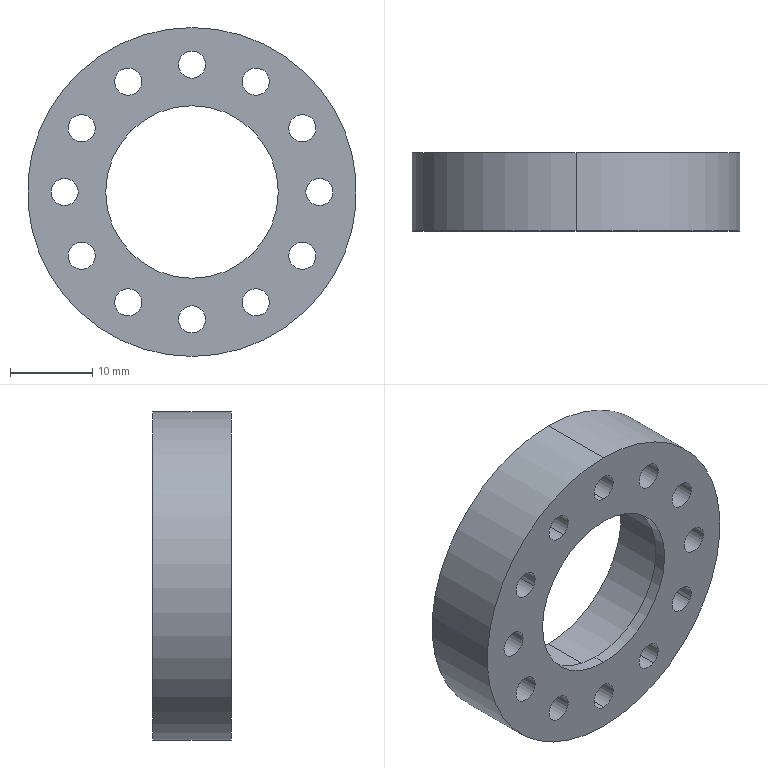Part | SolidWorks | mm | 1 solid | 33 faces | box 40 x 9.5 x 40 mm | volume 6516 mm3 | cylinder 30 | plane 3 | commonest cylinder face diameters 3.3 x24 21 x2 25 x2 40 x2
build123d program:
from build123d import *

# Parameters (mm, degrees)
SKETCH1_R           = 20
BOSS_EXTRUDE1_DEPTH = 9.5
SKETCH2_R           = 10
BOSS_EXTRUDE2_DEPTH = 7
SKETCH3_R           = 12.5
CUT_EXTRUDE1_DEPTH  = 8
SKETCH4_R           = 10.5
CUT_EXTRUDE2_DEPTH  = 30.394
M4_TAPPED_HOLE1_D   = 3.3
CIRPATTERN1_COUNT   = 12


with BuildPart() as part:
    # Sketch1 → Boss-Extrude1 (new body)
    with BuildSketch(Plane(origin=(0, 0, 0), x_dir=(1, 0, 0), z_dir=(0, 1, 0))):
        with Locations(Location((0, 0, 0), (0, 0, 270))):
            Circle(SKETCH1_R)
    extrude(amount=BOSS_EXTRUDE1_DEPTH)

    # Sketch2 → Boss-Extrude2 (add)
    with BuildSketch(Plane(origin=(0, 9.5, 0), x_dir=(1, 0, 0), z_dir=(0, 1, 0))):
        Circle(SKETCH2_R)
    extrude(amount=-BOSS_EXTRUDE2_DEPTH)

    # Sketch3 → Cut-Extrude1 (cut)
    with BuildSketch(Plane(origin=(0, 9.5, 0), x_dir=(1, 0, 0), z_dir=(0, 1, 0))):
        with Locations(Location((0, 0, 0), (0, 0, 270))):
            Circle(SKETCH3_R)
    extrude(amount=-CUT_EXTRUDE1_DEPTH, mode=Mode.SUBTRACT)

    # Sketch4 → Cut-Extrude2 (cut, through all)
    with BuildSketch(Plane(origin=(0, 1.5, 0), x_dir=(1, 0, 0), z_dir=(0, 1, 0))):
        with Locations(Location((0, 0, 0), (0, 0, 270))):
            Circle(SKETCH4_R)
    extrude(amount=-CUT_EXTRUDE2_DEPTH, mode=Mode.SUBTRACT)

    # M4 Tapped Hole1 (through all)
    with Locations(Plane(origin=(0, 0, 0), x_dir=(-1, 0, 0), z_dir=(0, -1, 0))):
        with Locations((0, -15.5)):
            m4_tapped_hole1 = Hole(M4_TAPPED_HOLE1_D / 2)

    # CirPattern1: M4 Tapped Hole1 ×12 about axis
    cirpattern1_axis = Axis((0, 0, 0), (0, 1, 0))
    for i in range(1, CIRPATTERN1_COUNT):
        add(m4_tapped_hole1.rotate(cirpattern1_axis, i * 360 / CIRPATTERN1_COUNT), mode=Mode.SUBTRACT)


solid = part.part
STEP:
#1=CARTESIAN_POINT('',(8.575,9.5,14.852));
#2=VERTEX_POINT('',#1);
#3=CARTESIAN_POINT('',(6.925,9.5,11.994));
#4=VERTEX_POINT('',#3);
#5=CARTESIAN_POINT('',(7.75,9.5,13.423));
#6=DIRECTION('',(0.,-1.,0.));
#7=DIRECTION('',(-0.5,0.,-0.866));
#8=AXIS2_PLACEMENT_3D('',#5,#6,#7);
#9=CIRCLE('',#8,1.65);
#10=EDGE_CURVE('',#2,#4,#9,.T.);
#11=ORIENTED_EDGE('',*,*,#10,.F.);
#12=CARTESIAN_POINT('',(8.575,-0.,14.852));
#13=VERTEX_POINT('',#12);
#14=CARTESIAN_POINT('',(8.575,0.,14.852));
#15=DIRECTION('',(0.,-1.,0.));
#16=VECTOR('',#15,1000.);
#17=LINE('',#14,#16);
#18=EDGE_CURVE('',#2,#13,#17,.T.);
#19=ORIENTED_EDGE('',*,*,#18,.T.);
#20=CARTESIAN_POINT('',(6.925,-0.,11.994));
#21=VERTEX_POINT('',#20);
#22=CARTESIAN_POINT('',(7.75,-0.,13.423));
#23=DIRECTION('',(0.,-1.,0.));
#24=DIRECTION('',(-0.5,0.,-0.866));
#25=AXIS2_PLACEMENT_3D('',#22,#23,#24);
#26=CIRCLE('',#25,1.65);
#27=EDGE_CURVE('',#13,#21,#26,.T.);
#28=ORIENTED_EDGE('',*,*,#27,.T.);
#29=CARTESIAN_POINT('',(6.925,0.,11.994));
#30=DIRECTION('',(0.,-1.,0.));
#31=VECTOR('',#30,1000.);
#32=LINE('',#29,#31);
#33=EDGE_CURVE('',#4,#21,#32,.T.);
#34=ORIENTED_EDGE('',*,*,#33,.F.);
#35=EDGE_LOOP('',(#11,#19,#28,#34));
#36=FACE_OUTER_BOUND('',#35,.T.);
#37=CARTESIAN_POINT('',(7.75,0.,13.423));
#38=DIRECTION('',(0.,-1.,0.));
#39=DIRECTION('',(-0.5,0.,-0.866));
#40=AXIS2_PLACEMENT_3D('',#37,#38,#39);
#41=CYLINDRICAL_SURFACE('',#40,1.65);
#42=ADVANCED_FACE('',(#36),#41,.F.);
#43=CARTESIAN_POINT('',(14.852,9.5,8.575));
#44=VERTEX_POINT('',#43);
#45=CARTESIAN_POINT('',(11.994,9.5,6.925));
#46=VERTEX_POINT('',#45);
#47=CARTESIAN_POINT('',(13.423,9.5,7.75));
#48=DIRECTION('',(0.,-1.,0.));
#49=DIRECTION('',(-0.866,0.,-0.5));
#50=AXIS2_PLACEMENT_3D('',#47,#48,#49);
#51=CIRCLE('',#50,1.65);
#52=EDGE_CURVE('',#44,#46,#51,.T.);
#53=ORIENTED_EDGE('',*,*,#52,.F.);
#54=CARTESIAN_POINT('',(14.852,-0.,8.575));
#55=VERTEX_POINT('',#54);
#56=CARTESIAN_POINT('',(14.852,0.,8.575));
#57=DIRECTION('',(0.,-1.,0.));
#58=VECTOR('',#57,1000.);
#59=LINE('',#56,#58);
#60=EDGE_CURVE('',#44,#55,#59,.T.);
#61=ORIENTED_EDGE('',*,*,#60,.T.);
#62=CARTESIAN_POINT('',(11.994,-0.,6.925));
#63=VERTEX_POINT('',#62);
#64=CARTESIAN_POINT('',(13.423,-0.,7.75));
#65=DIRECTION('',(0.,-1.,0.));
#66=DIRECTION('',(-0.866,0.,-0.5));
#67=AXIS2_PLACEMENT_3D('',#64,#65,#66);
#68=CIRCLE('',#67,1.65);
#69=EDGE_CURVE('',#55,#63,#68,.T.);
#70=ORIENTED_EDGE('',*,*,#69,.T.);
#71=CARTESIAN_POINT('',(11.994,0.,6.925));
#72=DIRECTION('',(0.,-1.,0.));
#73=VECTOR('',#72,1000.);
#74=LINE('',#71,#73);
#75=EDGE_CURVE('',#46,#63,#74,.T.);
#76=ORIENTED_EDGE('',*,*,#75,.F.);
#77=EDGE_LOOP('',(#53,#61,#70,#76));
#78=FACE_OUTER_BOUND('',#77,.T.);
#79=CARTESIAN_POINT('',(13.423,0.,7.75));
#80=DIRECTION('',(0.,-1.,0.));
#81=DIRECTION('',(-0.866,0.,-0.5));
#82=AXIS2_PLACEMENT_3D('',#79,#80,#81);
#83=CYLINDRICAL_SURFACE('',#82,1.65);
#84=ADVANCED_FACE('',(#78),#83,.F.);
#85=CARTESIAN_POINT('',(17.15,9.5,0.));
#86=VERTEX_POINT('',#85);
#87=CARTESIAN_POINT('',(13.85,9.5,0.));
#88=VERTEX_POINT('',#87);
#89=CARTESIAN_POINT('',(15.5,9.5,0.));
#90=DIRECTION('',(0.,-1.,0.));
#91=DIRECTION('',(-1.,0.,-0.));
#92=AXIS2_PLACEMENT_3D('',#89,#90,#91);
#93=CIRCLE('',#92,1.65);
#94=EDGE_CURVE('',#86,#88,#93,.T.);
#95=ORIENTED_EDGE('',*,*,#94,.F.);
#96=CARTESIAN_POINT('',(17.15,-0.,0.));
#97=VERTEX_POINT('',#96);
#98=CARTESIAN_POINT('',(17.15,0.,0.));
#99=DIRECTION('',(0.,-1.,0.));
#100=VECTOR('',#99,1000.);
#101=LINE('',#98,#100);
#102=EDGE_CURVE('',#86,#97,#101,.T.);
#103=ORIENTED_EDGE('',*,*,#102,.T.);
#104=CARTESIAN_POINT('',(13.85,-0.,0.));
#105=VERTEX_POINT('',#104);
#106=CARTESIAN_POINT('',(15.5,-0.,0.));
#107=DIRECTION('',(0.,-1.,0.));
#108=DIRECTION('',(-1.,0.,-0.));
#109=AXIS2_PLACEMENT_3D('',#106,#107,#108);
#110=CIRCLE('',#109,1.65);
#111=EDGE_CURVE('',#97,#105,#110,.T.);
#112=ORIENTED_EDGE('',*,*,#111,.T.);
#113=CARTESIAN_POINT('',(13.85,0.,0.));
#114=DIRECTION('',(0.,-1.,0.));
#115=VECTOR('',#114,1000.);
#116=LINE('',#113,#115);
#117=EDGE_CURVE('',#88,#105,#116,.T.);
#118=ORIENTED_EDGE('',*,*,#117,.F.);
#119=EDGE_LOOP('',(#95,#103,#112,#118));
#120=FACE_OUTER_BOUND('',#119,.T.);
#121=CARTESIAN_POINT('',(15.5,0.,0.));
#122=DIRECTION('',(0.,-1.,0.));
#123=DIRECTION('',(-1.,0.,-0.));
#124=AXIS2_PLACEMENT_3D('',#121,#122,#123);
#125=CYLINDRICAL_SURFACE('',#124,1.65);
#126=ADVANCED_FACE('',(#120),#125,.F.);
#127=CARTESIAN_POINT('',(14.852,9.5,-8.575));
#128=VERTEX_POINT('',#127);
#129=CARTESIAN_POINT('',(11.994,9.5,-6.925));
#130=VERTEX_POINT('',#129);
#131=CARTESIAN_POINT('',(13.423,9.5,-7.75));
#132=DIRECTION('',(0.,-1.,0.));
#133=DIRECTION('',(-0.866,0.,0.5));
#134=AXIS2_PLACEMENT_3D('',#131,#132,#133);
#135=CIRCLE('',#134,1.65);
#136=EDGE_CURVE('',#128,#130,#135,.T.);
#137=ORIENTED_EDGE('',*,*,#136,.F.);
#138=CARTESIAN_POINT('',(14.852,-0.,-8.575));
#139=VERTEX_POINT('',#138);
#140=CARTESIAN_POINT('',(14.852,0.,-8.575));
#141=DIRECTION('',(0.,-1.,0.));
#142=VECTOR('',#141,1000.);
#143=LINE('',#140,#142);
#144=EDGE_CURVE('',#128,#139,#143,.T.);
#145=ORIENTED_EDGE('',*,*,#144,.T.);
#146=CARTESIAN_POINT('',(11.994,-0.,-6.925));
#147=VERTEX_POINT('',#146);
#148=CARTESIAN_POINT('',(13.423,-0.,-7.75));
#149=DIRECTION('',(0.,-1.,0.));
#150=DIRECTION('',(-0.866,0.,0.5));
#151=AXIS2_PLACEMENT_3D('',#148,#149,#150);
#152=CIRCLE('',#151,1.65);
#153=EDGE_CURVE('',#139,#147,#152,.T.);
#154=ORIENTED_EDGE('',*,*,#153,.T.);
#155=CARTESIAN_POINT('',(11.994,0.,-6.925));
#156=DIRECTION('',(0.,-1.,0.));
#157=VECTOR('',#156,1000.);
#158=LINE('',#155,#157);
#159=EDGE_CURVE('',#130,#147,#158,.T.);
#160=ORIENTED_EDGE('',*,*,#159,.F.);
#161=EDGE_LOOP('',(#137,#145,#154,#160));
#162=FACE_OUTER_BOUND('',#161,.T.);
#163=CARTESIAN_POINT('',(13.423,0.,-7.75));
#164=DIRECTION('',(0.,-1.,0.));
#165=DIRECTION('',(-0.866,0.,0.5));
#166=AXIS2_PLACEMENT_3D('',#163,#164,#165);
#167=CYLINDRICAL_SURFACE('',#166,1.65);
#168=ADVANCED_FACE('',(#162),#167,.F.);
#169=CARTESIAN_POINT('',(8.575,9.5,-14.852));
#170=VERTEX_POINT('',#169);
#171=CARTESIAN_POINT('',(6.925,9.5,-11.994));
#172=VERTEX_POINT('',#171);
#173=CARTESIAN_POINT('',(7.75,9.5,-13.423));
#174=DIRECTION('',(0.,-1.,0.));
#175=DIRECTION('',(-0.5,0.,0.866));
#176=AXIS2_PLACEMENT_3D('',#173,#174,#175);
#177=CIRCLE('',#176,1.65);
#178=EDGE_CURVE('',#170,#172,#177,.T.);
#179=ORIENTED_EDGE('',*,*,#178,.F.);
#180=CARTESIAN_POINT('',(8.575,-0.,-14.852));
#181=VERTEX_POINT('',#180);
#182=CARTESIAN_POINT('',(8.575,0.,-14.852));
#183=DIRECTION('',(0.,-1.,0.));
#184=VECTOR('',#183,1000.);
#185=LINE('',#182,#184);
#186=EDGE_CURVE('',#170,#181,#185,.T.);
#187=ORIENTED_EDGE('',*,*,#186,.T.);
#188=CARTESIAN_POINT('',(6.925,-0.,-11.994));
#189=VERTEX_POINT('',#188);
#190=CARTESIAN_POINT('',(7.75,-0.,-13.423));
#191=DIRECTION('',(0.,-1.,0.));
#192=DIRECTION('',(-0.5,0.,0.866));
#193=AXIS2_PLACEMENT_3D('',#190,#191,#192);
#194=CIRCLE('',#193,1.65);
#195=EDGE_CURVE('',#181,#189,#194,.T.);
#196=ORIENTED_EDGE('',*,*,#195,.T.);
#197=CARTESIAN_POINT('',(6.925,0.,-11.994));
#198=DIRECTION('',(0.,-1.,0.));
#199=VECTOR('',#198,1000.);
#200=LINE('',#197,#199);
#201=EDGE_CURVE('',#172,#189,#200,.T.);
#202=ORIENTED_EDGE('',*,*,#201,.F.);
#203=EDGE_LOOP('',(#179,#187,#196,#202));
#204=FACE_OUTER_BOUND('',#203,.T.);
#205=CARTESIAN_POINT('',(7.75,0.,-13.423));
#206=DIRECTION('',(0.,-1.,0.));
#207=DIRECTION('',(-0.5,0.,0.866));
#208=AXIS2_PLACEMENT_3D('',#205,#206,#207);
#209=CYLINDRICAL_SURFACE('',#208,1.65);
#210=ADVANCED_FACE('',(#204),#209,.F.);
#211=CARTESIAN_POINT('',(0.,9.5,-17.15));
#212=VERTEX_POINT('',#211);
#213=CARTESIAN_POINT('',(0.,9.5,-13.85));
#214=VERTEX_POINT('',#213);
#215=CARTESIAN_POINT('',(0.,9.5,-15.5));
#216=DIRECTION('',(0.,-1.,0.));
#217=DIRECTION('',(0.,0.,1.));
#218=AXIS2_PLACEMENT_3D('',#215,#216,#217);
#219=CIRCLE('',#218,1.65);
#220=EDGE_CURVE('',#212,#214,#219,.T.);
#221=ORIENTED_EDGE('',*,*,#220,.F.);
#222=CARTESIAN_POINT('',(0.,-0.,-17.15));
#223=VERTEX_POINT('',#222);
#224=CARTESIAN_POINT('',(0.,0.,-17.15));
#225=DIRECTION('',(0.,-1.,0.));
#226=VECTOR('',#225,1000.);
#227=LINE('',#224,#226);
#228=EDGE_CURVE('',#212,#223,#227,.T.);
#229=ORIENTED_EDGE('',*,*,#228,.T.);
#230=CARTESIAN_POINT('',(0.,-0.,-13.85));
#231=VERTEX_POINT('',#230);
#232=CARTESIAN_POINT('',(0.,-0.,-15.5));
#233=DIRECTION('',(0.,-1.,0.));
#234=DIRECTION('',(0.,0.,1.));
#235=AXIS2_PLACEMENT_3D('',#232,#233,#234);
#236=CIRCLE('',#235,1.65);
#237=EDGE_CURVE('',#223,#231,#236,.T.);
#238=ORIENTED_EDGE('',*,*,#237,.T.);
#239=CARTESIAN_POINT('',(0.,0.,-13.85));
#240=DIRECTION('',(0.,-1.,0.));
#241=VECTOR('',#240,1000.);
#242=LINE('',#239,#241);
#243=EDGE_CURVE('',#214,#231,#242,.T.);
#244=ORIENTED_EDGE('',*,*,#243,.F.);
#245=EDGE_LOOP('',(#221,#229,#238,#244));
#246=FACE_OUTER_BOUND('',#245,.T.);
#247=CARTESIAN_POINT('',(0.,0.,-15.5));
#248=DIRECTION('',(0.,-1.,0.));
#249=DIRECTION('',(0.,0.,1.));
#250=AXIS2_PLACEMENT_3D('',#247,#248,#249);
#251=CYLINDRICAL_SURFACE('',#250,1.65);
#252=ADVANCED_FACE('',(#246),#251,.F.);
#253=CARTESIAN_POINT('',(-8.575,9.5,-14.852));
#254=VERTEX_POINT('',#253);
#255=CARTESIAN_POINT('',(-6.925,9.5,-11.994));
#256=VERTEX_POINT('',#255);
#257=CARTESIAN_POINT('',(-7.75,9.5,-13.423));
#258=DIRECTION('',(0.,-1.,0.));
#259=DIRECTION('',(0.5,0.,0.866));
#260=AXIS2_PLACEMENT_3D('',#257,#258,#259);
#261=CIRCLE('',#260,1.65);
#262=EDGE_CURVE('',#254,#256,#261,.T.);
#263=ORIENTED_EDGE('',*,*,#262,.F.);
#264=CARTESIAN_POINT('',(-8.575,-0.,-14.852));
#265=VERTEX_POINT('',#264);
#266=CARTESIAN_POINT('',(-8.575,0.,-14.852));
#267=DIRECTION('',(0.,-1.,0.));
#268=VECTOR('',#267,1000.);
#269=LINE('',#266,#268);
#270=EDGE_CURVE('',#254,#265,#269,.T.);
#271=ORIENTED_EDGE('',*,*,#270,.T.);
#272=CARTESIAN_POINT('',(-6.925,-0.,-11.994));
#273=VERTEX_POINT('',#272);
#274=CARTESIAN_POINT('',(-7.75,-0.,-13.423));
#275=DIRECTION('',(0.,-1.,0.));
#276=DIRECTION('',(0.5,0.,0.866));
#277=AXIS2_PLACEMENT_3D('',#274,#275,#276);
#278=CIRCLE('',#277,1.65);
#279=EDGE_CURVE('',#265,#273,#278,.T.);
#280=ORIENTED_EDGE('',*,*,#279,.T.);
#281=CARTESIAN_POINT('',(-6.925,0.,-11.994));
#282=DIRECTION('',(0.,-1.,0.));
#283=VECTOR('',#282,1000.);
#284=LINE('',#281,#283);
#285=EDGE_CURVE('',#256,#273,#284,.T.);
#286=ORIENTED_EDGE('',*,*,#285,.F.);
#287=EDGE_LOOP('',(#263,#271,#280,#286));
#288=FACE_OUTER_BOUND('',#287,.T.);
#289=CARTESIAN_POINT('',(-7.75,0.,-13.423));
#290=DIRECTION('',(0.,-1.,0.));
#291=DIRECTION('',(0.5,0.,0.866));
#292=AXIS2_PLACEMENT_3D('',#289,#290,#291);
#293=CYLINDRICAL_SURFACE('',#292,1.65);
#294=ADVANCED_FACE('',(#288),#293,.F.);
#295=CARTESIAN_POINT('',(-14.852,9.5,-8.575));
#296=VERTEX_POINT('',#295);
#297=CARTESIAN_POINT('',(-11.994,9.5,-6.925));
#298=VERTEX_POINT('',#297);
#299=CARTESIAN_POINT('',(-13.423,9.5,-7.75));
#300=DIRECTION('',(0.,-1.,0.));
#301=DIRECTION('',(0.866,0.,0.5));
#302=AXIS2_PLACEMENT_3D('',#299,#300,#301);
#303=CIRCLE('',#302,1.65);
#304=EDGE_CURVE('',#296,#298,#303,.T.);
#305=ORIENTED_EDGE('',*,*,#304,.F.);
#306=CARTESIAN_POINT('',(-14.852,-0.,-8.575));
#307=VERTEX_POINT('',#306);
#308=CARTESIAN_POINT('',(-14.852,0.,-8.575));
#309=DIRECTION('',(0.,-1.,0.));
#310=VECTOR('',#309,1000.);
#311=LINE('',#308,#310);
#312=EDGE_CURVE('',#296,#307,#311,.T.);
#313=ORIENTED_EDGE('',*,*,#312,.T.);
#314=CARTESIAN_POINT('',(-11.994,-0.,-6.925));
#315=VERTEX_POINT('',#314);
#316=CARTESIAN_POINT('',(-13.423,-0.,-7.75));
#317=DIRECTION('',(0.,-1.,0.));
#318=DIRECTION('',(0.866,0.,0.5));
#319=AXIS2_PLACEMENT_3D('',#316,#317,#318);
#320=CIRCLE('',#319,1.65);
#321=EDGE_CURVE('',#307,#315,#320,.T.);
#322=ORIENTED_EDGE('',*,*,#321,.T.);
#323=CARTESIAN_POINT('',(-11.994,0.,-6.925));
#324=DIRECTION('',(0.,-1.,0.));
#325=VECTOR('',#324,1000.);
#326=LINE('',#323,#325);
#327=EDGE_CURVE('',#298,#315,#326,.T.);
#328=ORIENTED_EDGE('',*,*,#327,.F.);
#329=EDGE_LOOP('',(#305,#313,#322,#328));
#330=FACE_OUTER_BOUND('',#329,.T.);
#331=CARTESIAN_POINT('',(-13.423,0.,-7.75));
#332=DIRECTION('',(0.,-1.,0.));
#333=DIRECTION('',(0.866,0.,0.5));
#334=AXIS2_PLACEMENT_3D('',#331,#332,#333);
#335=CYLINDRICAL_SURFACE('',#334,1.65);
#336=ADVANCED_FACE('',(#330),#335,.F.);
#337=CARTESIAN_POINT('',(-17.15,9.5,-0.));
#338=VERTEX_POINT('',#337);
#339=CARTESIAN_POINT('',(-13.85,9.5,-0.));
#340=VERTEX_POINT('',#339);
#341=CARTESIAN_POINT('',(-15.5,9.5,-0.));
#342=DIRECTION('',(0.,-1.,0.));
#343=DIRECTION('',(1.,0.,0.));
#344=AXIS2_PLACEMENT_3D('',#341,#342,#343);
#345=CIRCLE('',#344,1.65);
#346=EDGE_CURVE('',#338,#340,#345,.T.);
#347=ORIENTED_EDGE('',*,*,#346,.F.);
#348=CARTESIAN_POINT('',(-17.15,-0.,-0.));
#349=VERTEX_POINT('',#348);
#350=CARTESIAN_POINT('',(-17.15,0.,-0.));
#351=DIRECTION('',(0.,-1.,0.));
#352=VECTOR('',#351,1000.);
#353=LINE('',#350,#352);
#354=EDGE_CURVE('',#338,#349,#353,.T.);
#355=ORIENTED_EDGE('',*,*,#354,.T.);
#356=CARTESIAN_POINT('',(-13.85,-0.,-0.));
#357=VERTEX_POINT('',#356);
#358=CARTESIAN_POINT('',(-15.5,-0.,-0.));
#359=DIRECTION('',(0.,-1.,0.));
#360=DIRECTION('',(1.,0.,0.));
#361=AXIS2_PLACEMENT_3D('',#358,#359,#360);
#362=CIRCLE('',#361,1.65);
#363=EDGE_CURVE('',#349,#357,#362,.T.);
#364=ORIENTED_EDGE('',*,*,#363,.T.);
#365=CARTESIAN_POINT('',(-13.85,0.,-0.));
#366=DIRECTION('',(0.,-1.,0.));
#367=VECTOR('',#366,1000.);
#368=LINE('',#365,#367);
#369=EDGE_CURVE('',#340,#357,#368,.T.);
#370=ORIENTED_EDGE('',*,*,#369,.F.);
#371=EDGE_LOOP('',(#347,#355,#364,#370));
#372=FACE_OUTER_BOUND('',#371,.T.);
#373=CARTESIAN_POINT('',(-15.5,0.,-0.));
#374=DIRECTION('',(0.,-1.,0.));
#375=DIRECTION('',(1.,0.,0.));
#376=AXIS2_PLACEMENT_3D('',#373,#374,#375);
#377=CYLINDRICAL_SURFACE('',#376,1.65);
#378=ADVANCED_FACE('',(#372),#377,.F.);
#379=CARTESIAN_POINT('',(-14.852,9.5,8.575));
#380=VERTEX_POINT('',#379);
#381=CARTESIAN_POINT('',(-11.994,9.5,6.925));
#382=VERTEX_POINT('',#381);
#383=CARTESIAN_POINT('',(-13.423,9.5,7.75));
#384=DIRECTION('',(0.,-1.,0.));
#385=DIRECTION('',(0.866,0.,-0.5));
#386=AXIS2_PLACEMENT_3D('',#383,#384,#385);
#387=CIRCLE('',#386,1.65);
#388=EDGE_CURVE('',#380,#382,#387,.T.);
#389=ORIENTED_EDGE('',*,*,#388,.F.);
#390=CARTESIAN_POINT('',(-14.852,-0.,8.575));
#391=VERTEX_POINT('',#390);
#392=CARTESIAN_POINT('',(-14.852,0.,8.575));
#393=DIRECTION('',(0.,-1.,0.));
#394=VECTOR('',#393,1000.);
#395=LINE('',#392,#394);
#396=EDGE_CURVE('',#380,#391,#395,.T.);
#397=ORIENTED_EDGE('',*,*,#396,.T.);
#398=CARTESIAN_POINT('',(-11.994,-0.,6.925));
#399=VERTEX_POINT('',#398);
#400=CARTESIAN_POINT('',(-13.423,-0.,7.75));
#401=DIRECTION('',(0.,-1.,0.));
#402=DIRECTION('',(0.866,0.,-0.5));
#403=AXIS2_PLACEMENT_3D('',#400,#401,#402);
#404=CIRCLE('',#403,1.65);
#405=EDGE_CURVE('',#391,#399,#404,.T.);
#406=ORIENTED_EDGE('',*,*,#405,.T.);
#407=CARTESIAN_POINT('',(-11.994,0.,6.925));
#408=DIRECTION('',(0.,-1.,0.));
#409=VECTOR('',#408,1000.);
#410=LINE('',#407,#409);
#411=EDGE_CURVE('',#382,#399,#410,.T.);
#412=ORIENTED_EDGE('',*,*,#411,.F.);
#413=EDGE_LOOP('',(#389,#397,#406,#412));
#414=FACE_OUTER_BOUND('',#413,.T.);
#415=CARTESIAN_POINT('',(-13.423,0.,7.75));
#416=DIRECTION('',(0.,-1.,0.));
#417=DIRECTION('',(0.866,0.,-0.5));
#418=AXIS2_PLACEMENT_3D('',#415,#416,#417);
#419=CYLINDRICAL_SURFACE('',#418,1.65);
#420=ADVANCED_FACE('',(#414),#419,.F.);
#421=CARTESIAN_POINT('',(-8.575,9.5,14.852));
#422=VERTEX_POINT('',#421);
#423=CARTESIAN_POINT('',(-6.925,9.5,11.994));
#424=VERTEX_POINT('',#423);
#425=CARTESIAN_POINT('',(-7.75,9.5,13.423));
#426=DIRECTION('',(0.,-1.,0.));
#427=DIRECTION('',(0.5,0.,-0.866));
#428=AXIS2_PLACEMENT_3D('',#425,#426,#427);
#429=CIRCLE('',#428,1.65);
#430=EDGE_CURVE('',#422,#424,#429,.T.);
#431=ORIENTED_EDGE('',*,*,#430,.F.);
#432=CARTESIAN_POINT('',(-8.575,-0.,14.852));
#433=VERTEX_POINT('',#432);
#434=CARTESIAN_POINT('',(-8.575,0.,14.852));
#435=DIRECTION('',(0.,-1.,0.));
#436=VECTOR('',#435,1000.);
#437=LINE('',#434,#436);
#438=EDGE_CURVE('',#422,#433,#437,.T.);
#439=ORIENTED_EDGE('',*,*,#438,.T.);
#440=CARTESIAN_POINT('',(-6.925,-0.,11.994));
#441=VERTEX_POINT('',#440);
#442=CARTESIAN_POINT('',(-7.75,-0.,13.423));
#443=DIRECTION('',(0.,-1.,0.));
#444=DIRECTION('',(0.5,0.,-0.866));
#445=AXIS2_PLACEMENT_3D('',#442,#443,#444);
#446=CIRCLE('',#445,1.65);
#447=EDGE_CURVE('',#433,#441,#446,.T.);
#448=ORIENTED_EDGE('',*,*,#447,.T.);
#449=CARTESIAN_POINT('',(-6.925,0.,11.994));
#450=DIRECTION('',(0.,-1.,0.));
#451=VECTOR('',#450,1000.);
#452=LINE('',#449,#451);
#453=EDGE_CURVE('',#424,#441,#452,.T.);
#454=ORIENTED_EDGE('',*,*,#453,.F.);
#455=EDGE_LOOP('',(#431,#439,#448,#454));
#456=FACE_OUTER_BOUND('',#455,.T.);
#457=CARTESIAN_POINT('',(-7.75,0.,13.423));
#458=DIRECTION('',(0.,-1.,0.));
#459=DIRECTION('',(0.5,0.,-0.866));
#460=AXIS2_PLACEMENT_3D('',#457,#458,#459);
#461=CYLINDRICAL_SURFACE('',#460,1.65);
#462=ADVANCED_FACE('',(#456),#461,.F.);
#463=CARTESIAN_POINT('',(-0.,9.5,17.15));
#464=VERTEX_POINT('',#463);
#465=CARTESIAN_POINT('',(-0.,9.5,13.85));
#466=VERTEX_POINT('',#465);
#467=CARTESIAN_POINT('',(-0.,9.5,15.5));
#468=DIRECTION('',(0.,-1.,0.));
#469=DIRECTION('',(0.,0.,-1.));
#470=AXIS2_PLACEMENT_3D('',#467,#468,#469);
#471=CIRCLE('',#470,1.65);
#472=EDGE_CURVE('',#464,#466,#471,.T.);
#473=ORIENTED_EDGE('',*,*,#472,.F.);
#474=CARTESIAN_POINT('',(-0.,-0.,17.15));
#475=VERTEX_POINT('',#474);
#476=CARTESIAN_POINT('',(-0.,0.,17.15));
#477=DIRECTION('',(0.,-1.,0.));
#478=VECTOR('',#477,1000.);
#479=LINE('',#476,#478);
#480=EDGE_CURVE('',#464,#475,#479,.T.);
#481=ORIENTED_EDGE('',*,*,#480,.T.);
#482=CARTESIAN_POINT('',(-0.,-0.,13.85));
#483=VERTEX_POINT('',#482);
#484=CARTESIAN_POINT('',(-0.,-0.,15.5));
#485=DIRECTION('',(0.,-1.,0.));
#486=DIRECTION('',(0.,0.,-1.));
#487=AXIS2_PLACEMENT_3D('',#484,#485,#486);
#488=CIRCLE('',#487,1.65);
#489=EDGE_CURVE('',#475,#483,#488,.T.);
#490=ORIENTED_EDGE('',*,*,#489,.T.);
#491=CARTESIAN_POINT('',(-0.,0.,13.85));
#492=DIRECTION('',(0.,-1.,0.));
#493=VECTOR('',#492,1000.);
#494=LINE('',#491,#493);
#495=EDGE_CURVE('',#466,#483,#494,.T.);
#496=ORIENTED_EDGE('',*,*,#495,.F.);
#497=EDGE_LOOP('',(#473,#481,#490,#496));
#498=FACE_OUTER_BOUND('',#497,.T.);
#499=CARTESIAN_POINT('',(-0.,0.,15.5));
#500=DIRECTION('',(0.,-1.,0.));
#501=DIRECTION('',(0.,0.,-1.));
#502=AXIS2_PLACEMENT_3D('',#499,#500,#501);
#503=CYLINDRICAL_SURFACE('',#502,1.65);
#504=ADVANCED_FACE('',(#498),#503,.F.);
#505=CARTESIAN_POINT('',(0.,0.,-10.5));
#506=VERTEX_POINT('',#505);
#507=CARTESIAN_POINT('',(0.,0.,10.5));
#508=VERTEX_POINT('',#507);
#509=CARTESIAN_POINT('',(0.,0.,0.));
#510=DIRECTION('',(0.,1.,0.));
#511=DIRECTION('',(0.,0.,1.));
#512=AXIS2_PLACEMENT_3D('',#509,#510,#511);
#513=CIRCLE('',#512,10.5);
#514=EDGE_CURVE('',#506,#508,#513,.T.);
#515=ORIENTED_EDGE('',*,*,#514,.F.);
#516=CARTESIAN_POINT('',(0.,1.5,-10.5));
#517=VERTEX_POINT('',#516);
#518=CARTESIAN_POINT('',(0.,0.,-10.5));
#519=DIRECTION('',(0.,1.,0.));
#520=VECTOR('',#519,1000.);
#521=LINE('',#518,#520);
#522=EDGE_CURVE('',#506,#517,#521,.T.);
#523=ORIENTED_EDGE('',*,*,#522,.T.);
#524=CARTESIAN_POINT('',(0.,1.5,10.5));
#525=VERTEX_POINT('',#524);
#526=CARTESIAN_POINT('',(0.,1.5,0.));
#527=DIRECTION('',(0.,1.,0.));
#528=DIRECTION('',(0.,0.,1.));
#529=AXIS2_PLACEMENT_3D('',#526,#527,#528);
#530=CIRCLE('',#529,10.5);
#531=EDGE_CURVE('',#517,#525,#530,.T.);
#532=ORIENTED_EDGE('',*,*,#531,.T.);
#533=CARTESIAN_POINT('',(0.,0.,10.5));
#534=DIRECTION('',(0.,1.,0.));
#535=VECTOR('',#534,1000.);
#536=LINE('',#533,#535);
#537=EDGE_CURVE('',#508,#525,#536,.T.);
#538=ORIENTED_EDGE('',*,*,#537,.F.);
#539=EDGE_LOOP('',(#515,#523,#532,#538));
#540=FACE_OUTER_BOUND('',#539,.T.);
#541=CARTESIAN_POINT('',(0.,0.,0.));
#542=DIRECTION('',(0.,1.,0.));
#543=DIRECTION('',(0.,0.,1.));
#544=AXIS2_PLACEMENT_3D('',#541,#542,#543);
#545=CYLINDRICAL_SURFACE('',#544,10.5);
#546=ADVANCED_FACE('',(#540),#545,.F.);
#547=CARTESIAN_POINT('',(0.,1.5,-12.5));
#548=VERTEX_POINT('',#547);
#549=CARTESIAN_POINT('',(0.,1.5,12.5));
#550=VERTEX_POINT('',#549);
#551=CARTESIAN_POINT('',(0.,1.5,0.));
#552=DIRECTION('',(0.,1.,0.));
#553=DIRECTION('',(0.,0.,1.));
#554=AXIS2_PLACEMENT_3D('',#551,#552,#553);
#555=CIRCLE('',#554,12.5);
#556=EDGE_CURVE('',#548,#550,#555,.T.);
#557=ORIENTED_EDGE('',*,*,#556,.F.);
#558=CARTESIAN_POINT('',(0.,9.5,-12.5));
#559=VERTEX_POINT('',#558);
#560=CARTESIAN_POINT('',(0.,1.5,-12.5));
#561=DIRECTION('',(0.,1.,0.));
#562=VECTOR('',#561,1000.);
#563=LINE('',#560,#562);
#564=EDGE_CURVE('',#548,#559,#563,.T.);
#565=ORIENTED_EDGE('',*,*,#564,.T.);
#566=CARTESIAN_POINT('',(0.,9.5,12.5));
#567=VERTEX_POINT('',#566);
#568=CARTESIAN_POINT('',(0.,9.5,0.));
#569=DIRECTION('',(0.,1.,0.));
#570=DIRECTION('',(0.,0.,1.));
#571=AXIS2_PLACEMENT_3D('',#568,#569,#570);
#572=CIRCLE('',#571,12.5);
#573=EDGE_CURVE('',#559,#567,#572,.T.);
#574=ORIENTED_EDGE('',*,*,#573,.T.);
#575=CARTESIAN_POINT('',(0.,1.5,12.5));
#576=DIRECTION('',(0.,1.,0.));
#577=VECTOR('',#576,1000.);
#578=LINE('',#575,#577);
#579=EDGE_CURVE('',#550,#567,#578,.T.);
#580=ORIENTED_EDGE('',*,*,#579,.F.);
#581=EDGE_LOOP('',(#557,#565,#574,#580));
#582=FACE_OUTER_BOUND('',#581,.T.);
#583=CARTESIAN_POINT('',(0.,1.5,0.));
#584=DIRECTION('',(0.,1.,0.));
#585=DIRECTION('',(0.,0.,1.));
#586=AXIS2_PLACEMENT_3D('',#583,#584,#585);
#587=CYLINDRICAL_SURFACE('',#586,12.5);
#588=ADVANCED_FACE('',(#582),#587,.F.);
#589=CARTESIAN_POINT('',(0.,9.5,20.));
#590=VERTEX_POINT('',#589);
#591=CARTESIAN_POINT('',(0.,9.5,-20.));
#592=VERTEX_POINT('',#591);
#593=CARTESIAN_POINT('',(0.,9.5,0.));
#594=DIRECTION('',(0.,1.,0.));
#595=DIRECTION('',(0.,0.,1.));
#596=AXIS2_PLACEMENT_3D('',#593,#594,#595);
#597=CIRCLE('',#596,20.);
#598=EDGE_CURVE('',#590,#592,#597,.T.);
#599=ORIENTED_EDGE('',*,*,#598,.F.);
#600=CARTESIAN_POINT('',(0.,0.,20.));
#601=VERTEX_POINT('',#600);
#602=CARTESIAN_POINT('',(0.,9.5,20.));
#603=DIRECTION('',(0.,-1.,0.));
#604=VECTOR('',#603,1000.);
#605=LINE('',#602,#604);
#606=EDGE_CURVE('',#590,#601,#605,.T.);
#607=ORIENTED_EDGE('',*,*,#606,.T.);
#608=CARTESIAN_POINT('',(0.,0.,-20.));
#609=VERTEX_POINT('',#608);
#610=CARTESIAN_POINT('',(0.,0.,0.));
#611=DIRECTION('',(0.,1.,0.));
#612=DIRECTION('',(0.,0.,1.));
#613=AXIS2_PLACEMENT_3D('',#610,#611,#612);
#614=CIRCLE('',#613,20.);
#615=EDGE_CURVE('',#601,#609,#614,.T.);
#616=ORIENTED_EDGE('',*,*,#615,.T.);
#617=CARTESIAN_POINT('',(0.,9.5,-20.));
#618=DIRECTION('',(0.,-1.,0.));
#619=VECTOR('',#618,1000.);
#620=LINE('',#617,#619);
#621=EDGE_CURVE('',#592,#609,#620,.T.);
#622=ORIENTED_EDGE('',*,*,#621,.F.);
#623=EDGE_LOOP('',(#599,#607,#616,#622));
#624=FACE_OUTER_BOUND('',#623,.T.);
#625=CARTESIAN_POINT('',(0.,9.5,0.));
#626=DIRECTION('',(0.,-1.,0.));
#627=DIRECTION('',(0.,0.,-1.));
#628=AXIS2_PLACEMENT_3D('',#625,#626,#627);
#629=CYLINDRICAL_SURFACE('',#628,20.);
#630=ADVANCED_FACE('',(#624),#629,.T.);
#631=ORIENTED_EDGE('',*,*,#606,.F.);
#632=CARTESIAN_POINT('',(0.,9.5,0.));
#633=DIRECTION('',(0.,1.,0.));
#634=DIRECTION('',(0.,0.,1.));
#635=AXIS2_PLACEMENT_3D('',#632,#633,#634);
#636=CIRCLE('',#635,20.);
#637=EDGE_CURVE('',#592,#590,#636,.T.);
#638=ORIENTED_EDGE('',*,*,#637,.F.);
#639=ORIENTED_EDGE('',*,*,#621,.T.);
#640=CARTESIAN_POINT('',(0.,0.,0.));
#641=DIRECTION('',(0.,1.,0.));
#642=DIRECTION('',(0.,0.,1.));
#643=AXIS2_PLACEMENT_3D('',#640,#641,#642);
#644=CIRCLE('',#643,20.);
#645=EDGE_CURVE('',#609,#601,#644,.T.);
#646=ORIENTED_EDGE('',*,*,#645,.T.);
#647=EDGE_LOOP('',(#631,#638,#639,#646));
#648=FACE_OUTER_BOUND('',#647,.T.);
#649=CARTESIAN_POINT('',(0.,9.5,0.));
#650=DIRECTION('',(0.,-1.,0.));
#651=DIRECTION('',(0.,0.,-1.));
#652=AXIS2_PLACEMENT_3D('',#649,#650,#651);
#653=CYLINDRICAL_SURFACE('',#652,20.);
#654=ADVANCED_FACE('',(#648),#653,.T.);
#655=CARTESIAN_POINT('',(7.75,9.5,13.423));
#656=DIRECTION('',(0.,-1.,0.));
#657=DIRECTION('',(-0.5,0.,-0.866));
#658=AXIS2_PLACEMENT_3D('',#655,#656,#657);
#659=CIRCLE('',#658,1.65);
#660=EDGE_CURVE('',#4,#2,#659,.T.);
#661=ORIENTED_EDGE('',*,*,#660,.T.);
#662=ORIENTED_EDGE('',*,*,#10,.T.);
#663=EDGE_LOOP('',(#661,#662));
#664=FACE_BOUND('',#663,.T.);
#665=CARTESIAN_POINT('',(13.423,9.5,7.75));
#666=DIRECTION('',(0.,-1.,0.));
#667=DIRECTION('',(-0.866,0.,-0.5));
#668=AXIS2_PLACEMENT_3D('',#665,#666,#667);
#669=CIRCLE('',#668,1.65);
#670=EDGE_CURVE('',#46,#44,#669,.T.);
#671=ORIENTED_EDGE('',*,*,#670,.T.);
#672=ORIENTED_EDGE('',*,*,#52,.T.);
#673=EDGE_LOOP('',(#671,#672));
#674=FACE_BOUND('',#673,.T.);
#675=CARTESIAN_POINT('',(15.5,9.5,0.));
#676=DIRECTION('',(0.,-1.,0.));
#677=DIRECTION('',(-1.,0.,-0.));
#678=AXIS2_PLACEMENT_3D('',#675,#676,#677);
#679=CIRCLE('',#678,1.65);
#680=EDGE_CURVE('',#88,#86,#679,.T.);
#681=ORIENTED_EDGE('',*,*,#680,.T.);
#682=ORIENTED_EDGE('',*,*,#94,.T.);
#683=EDGE_LOOP('',(#681,#682));
#684=FACE_BOUND('',#683,.T.);
#685=CARTESIAN_POINT('',(13.423,9.5,-7.75));
#686=DIRECTION('',(0.,-1.,0.));
#687=DIRECTION('',(-0.866,0.,0.5));
#688=AXIS2_PLACEMENT_3D('',#685,#686,#687);
#689=CIRCLE('',#688,1.65);
#690=EDGE_CURVE('',#130,#128,#689,.T.);
#691=ORIENTED_EDGE('',*,*,#690,.T.);
#692=ORIENTED_EDGE('',*,*,#136,.T.);
#693=EDGE_LOOP('',(#691,#692));
#694=FACE_BOUND('',#693,.T.);
#695=CARTESIAN_POINT('',(7.75,9.5,-13.423));
#696=DIRECTION('',(0.,-1.,0.));
#697=DIRECTION('',(-0.5,0.,0.866));
#698=AXIS2_PLACEMENT_3D('',#695,#696,#697);
#699=CIRCLE('',#698,1.65);
#700=EDGE_CURVE('',#172,#170,#699,.T.);
#701=ORIENTED_EDGE('',*,*,#700,.T.);
#702=ORIENTED_EDGE('',*,*,#178,.T.);
#703=EDGE_LOOP('',(#701,#702));
#704=FACE_BOUND('',#703,.T.);
#705=CARTESIAN_POINT('',(0.,9.5,-15.5));
#706=DIRECTION('',(0.,-1.,0.));
#707=DIRECTION('',(0.,0.,1.));
#708=AXIS2_PLACEMENT_3D('',#705,#706,#707);
#709=CIRCLE('',#708,1.65);
#710=EDGE_CURVE('',#214,#212,#709,.T.);
#711=ORIENTED_EDGE('',*,*,#710,.T.);
#712=ORIENTED_EDGE('',*,*,#220,.T.);
#713=EDGE_LOOP('',(#711,#712));
#714=FACE_BOUND('',#713,.T.);
#715=CARTESIAN_POINT('',(-7.75,9.5,-13.423));
#716=DIRECTION('',(0.,-1.,0.));
#717=DIRECTION('',(0.5,0.,0.866));
#718=AXIS2_PLACEMENT_3D('',#715,#716,#717);
#719=CIRCLE('',#718,1.65);
#720=EDGE_CURVE('',#256,#254,#719,.T.);
#721=ORIENTED_EDGE('',*,*,#720,.T.);
#722=ORIENTED_EDGE('',*,*,#262,.T.);
#723=EDGE_LOOP('',(#721,#722));
#724=FACE_BOUND('',#723,.T.);
#725=CARTESIAN_POINT('',(-13.423,9.5,-7.75));
#726=DIRECTION('',(0.,-1.,0.));
#727=DIRECTION('',(0.866,0.,0.5));
#728=AXIS2_PLACEMENT_3D('',#725,#726,#727);
#729=CIRCLE('',#728,1.65);
#730=EDGE_CURVE('',#298,#296,#729,.T.);
#731=ORIENTED_EDGE('',*,*,#730,.T.);
#732=ORIENTED_EDGE('',*,*,#304,.T.);
#733=EDGE_LOOP('',(#731,#732));
#734=FACE_BOUND('',#733,.T.);
#735=CARTESIAN_POINT('',(-15.5,9.5,-0.));
#736=DIRECTION('',(0.,-1.,0.));
#737=DIRECTION('',(1.,0.,0.));
#738=AXIS2_PLACEMENT_3D('',#735,#736,#737);
#739=CIRCLE('',#738,1.65);
#740=EDGE_CURVE('',#340,#338,#739,.T.);
#741=ORIENTED_EDGE('',*,*,#740,.T.);
#742=ORIENTED_EDGE('',*,*,#346,.T.);
#743=EDGE_LOOP('',(#741,#742));
#744=FACE_BOUND('',#743,.T.);
#745=CARTESIAN_POINT('',(-13.423,9.5,7.75));
#746=DIRECTION('',(0.,-1.,0.));
#747=DIRECTION('',(0.866,0.,-0.5));
#748=AXIS2_PLACEMENT_3D('',#745,#746,#747);
#749=CIRCLE('',#748,1.65);
#750=EDGE_CURVE('',#382,#380,#749,.T.);
#751=ORIENTED_EDGE('',*,*,#750,.T.);
#752=ORIENTED_EDGE('',*,*,#388,.T.);
#753=EDGE_LOOP('',(#751,#752));
#754=FACE_BOUND('',#753,.T.);
#755=CARTESIAN_POINT('',(-7.75,9.5,13.423));
#756=DIRECTION('',(0.,-1.,0.));
#757=DIRECTION('',(0.5,0.,-0.866));
#758=AXIS2_PLACEMENT_3D('',#755,#756,#757);
#759=CIRCLE('',#758,1.65);
#760=EDGE_CURVE('',#424,#422,#759,.T.);
#761=ORIENTED_EDGE('',*,*,#760,.T.);
#762=ORIENTED_EDGE('',*,*,#430,.T.);
#763=EDGE_LOOP('',(#761,#762));
#764=FACE_BOUND('',#763,.T.);
#765=CARTESIAN_POINT('',(-0.,9.5,15.5));
#766=DIRECTION('',(0.,-1.,0.));
#767=DIRECTION('',(0.,0.,-1.));
#768=AXIS2_PLACEMENT_3D('',#765,#766,#767);
#769=CIRCLE('',#768,1.65);
#770=EDGE_CURVE('',#466,#464,#769,.T.);
#771=ORIENTED_EDGE('',*,*,#770,.T.);
#772=ORIENTED_EDGE('',*,*,#472,.T.);
#773=EDGE_LOOP('',(#771,#772));
#774=FACE_BOUND('',#773,.T.);
#775=CARTESIAN_POINT('',(0.,9.5,0.));
#776=DIRECTION('',(0.,1.,0.));
#777=DIRECTION('',(0.,0.,1.));
#778=AXIS2_PLACEMENT_3D('',#775,#776,#777);
#779=CIRCLE('',#778,12.5);
#780=EDGE_CURVE('',#567,#559,#779,.T.);
#781=ORIENTED_EDGE('',*,*,#780,.F.);
#782=ORIENTED_EDGE('',*,*,#573,.F.);
#783=EDGE_LOOP('',(#781,#782));
#784=FACE_BOUND('',#783,.T.);
#785=ORIENTED_EDGE('',*,*,#637,.T.);
#786=ORIENTED_EDGE('',*,*,#598,.T.);
#787=EDGE_LOOP('',(#785,#786));
#788=FACE_OUTER_BOUND('',#787,.T.);
#789=CARTESIAN_POINT('',(0.,9.5,0.));
#790=DIRECTION('',(0.,1.,0.));
#791=DIRECTION('',(0.,0.,1.));
#792=AXIS2_PLACEMENT_3D('',#789,#790,#791);
#793=PLANE('',#792);
#794=ADVANCED_FACE('',(#664,#674,#684,#694,#704,#714,#724,#734,#744,#754,#764,#774,#784,#788),#793,.T.);
#795=CARTESIAN_POINT('',(7.75,-0.,13.423));
#796=DIRECTION('',(0.,-1.,0.));
#797=DIRECTION('',(-0.5,0.,-0.866));
#798=AXIS2_PLACEMENT_3D('',#795,#796,#797);
#799=CIRCLE('',#798,1.65);
#800=EDGE_CURVE('',#21,#13,#799,.T.);
#801=ORIENTED_EDGE('',*,*,#800,.F.);
#802=ORIENTED_EDGE('',*,*,#27,.F.);
#803=EDGE_LOOP('',(#801,#802));
#804=FACE_BOUND('',#803,.T.);
#805=CARTESIAN_POINT('',(13.423,-0.,7.75));
#806=DIRECTION('',(0.,-1.,0.));
#807=DIRECTION('',(-0.866,0.,-0.5));
#808=AXIS2_PLACEMENT_3D('',#805,#806,#807);
#809=CIRCLE('',#808,1.65);
#810=EDGE_CURVE('',#63,#55,#809,.T.);
#811=ORIENTED_EDGE('',*,*,#810,.F.);
#812=ORIENTED_EDGE('',*,*,#69,.F.);
#813=EDGE_LOOP('',(#811,#812));
#814=FACE_BOUND('',#813,.T.);
#815=CARTESIAN_POINT('',(15.5,-0.,0.));
#816=DIRECTION('',(0.,-1.,0.));
#817=DIRECTION('',(-1.,0.,-0.));
#818=AXIS2_PLACEMENT_3D('',#815,#816,#817);
#819=CIRCLE('',#818,1.65);
#820=EDGE_CURVE('',#105,#97,#819,.T.);
#821=ORIENTED_EDGE('',*,*,#820,.F.);
#822=ORIENTED_EDGE('',*,*,#111,.F.);
#823=EDGE_LOOP('',(#821,#822));
#824=FACE_BOUND('',#823,.T.);
#825=CARTESIAN_POINT('',(13.423,-0.,-7.75));
#826=DIRECTION('',(0.,-1.,0.));
#827=DIRECTION('',(-0.866,0.,0.5));
#828=AXIS2_PLACEMENT_3D('',#825,#826,#827);
#829=CIRCLE('',#828,1.65);
#830=EDGE_CURVE('',#147,#139,#829,.T.);
#831=ORIENTED_EDGE('',*,*,#830,.F.);
#832=ORIENTED_EDGE('',*,*,#153,.F.);
#833=EDGE_LOOP('',(#831,#832));
#834=FACE_BOUND('',#833,.T.);
#835=CARTESIAN_POINT('',(7.75,-0.,-13.423));
#836=DIRECTION('',(0.,-1.,0.));
#837=DIRECTION('',(-0.5,0.,0.866));
#838=AXIS2_PLACEMENT_3D('',#835,#836,#837);
#839=CIRCLE('',#838,1.65);
#840=EDGE_CURVE('',#189,#181,#839,.T.);
#841=ORIENTED_EDGE('',*,*,#840,.F.);
#842=ORIENTED_EDGE('',*,*,#195,.F.);
#843=EDGE_LOOP('',(#841,#842));
#844=FACE_BOUND('',#843,.T.);
#845=CARTESIAN_POINT('',(0.,-0.,-15.5));
#846=DIRECTION('',(0.,-1.,0.));
#847=DIRECTION('',(0.,0.,1.));
#848=AXIS2_PLACEMENT_3D('',#845,#846,#847);
#849=CIRCLE('',#848,1.65);
#850=EDGE_CURVE('',#231,#223,#849,.T.);
#851=ORIENTED_EDGE('',*,*,#850,.F.);
#852=ORIENTED_EDGE('',*,*,#237,.F.);
#853=EDGE_LOOP('',(#851,#852));
#854=FACE_BOUND('',#853,.T.);
#855=CARTESIAN_POINT('',(-7.75,-0.,-13.423));
#856=DIRECTION('',(0.,-1.,0.));
#857=DIRECTION('',(0.5,0.,0.866));
#858=AXIS2_PLACEMENT_3D('',#855,#856,#857);
#859=CIRCLE('',#858,1.65);
#860=EDGE_CURVE('',#273,#265,#859,.T.);
#861=ORIENTED_EDGE('',*,*,#860,.F.);
#862=ORIENTED_EDGE('',*,*,#279,.F.);
#863=EDGE_LOOP('',(#861,#862));
#864=FACE_BOUND('',#863,.T.);
#865=CARTESIAN_POINT('',(-13.423,-0.,-7.75));
#866=DIRECTION('',(0.,-1.,0.));
#867=DIRECTION('',(0.866,0.,0.5));
#868=AXIS2_PLACEMENT_3D('',#865,#866,#867);
#869=CIRCLE('',#868,1.65);
#870=EDGE_CURVE('',#315,#307,#869,.T.);
#871=ORIENTED_EDGE('',*,*,#870,.F.);
#872=ORIENTED_EDGE('',*,*,#321,.F.);
#873=EDGE_LOOP('',(#871,#872));
#874=FACE_BOUND('',#873,.T.);
#875=CARTESIAN_POINT('',(-15.5,-0.,-0.));
#876=DIRECTION('',(0.,-1.,0.));
#877=DIRECTION('',(1.,0.,0.));
#878=AXIS2_PLACEMENT_3D('',#875,#876,#877);
#879=CIRCLE('',#878,1.65);
#880=EDGE_CURVE('',#357,#349,#879,.T.);
#881=ORIENTED_EDGE('',*,*,#880,.F.);
#882=ORIENTED_EDGE('',*,*,#363,.F.);
#883=EDGE_LOOP('',(#881,#882));
#884=FACE_BOUND('',#883,.T.);
#885=CARTESIAN_POINT('',(-13.423,-0.,7.75));
#886=DIRECTION('',(0.,-1.,0.));
#887=DIRECTION('',(0.866,0.,-0.5));
#888=AXIS2_PLACEMENT_3D('',#885,#886,#887);
#889=CIRCLE('',#888,1.65);
#890=EDGE_CURVE('',#399,#391,#889,.T.);
#891=ORIENTED_EDGE('',*,*,#890,.F.);
#892=ORIENTED_EDGE('',*,*,#405,.F.);
#893=EDGE_LOOP('',(#891,#892));
#894=FACE_BOUND('',#893,.T.);
#895=CARTESIAN_POINT('',(-7.75,-0.,13.423));
#896=DIRECTION('',(0.,-1.,0.));
#897=DIRECTION('',(0.5,0.,-0.866));
#898=AXIS2_PLACEMENT_3D('',#895,#896,#897);
#899=CIRCLE('',#898,1.65);
#900=EDGE_CURVE('',#441,#433,#899,.T.);
#901=ORIENTED_EDGE('',*,*,#900,.F.);
#902=ORIENTED_EDGE('',*,*,#447,.F.);
#903=EDGE_LOOP('',(#901,#902));
#904=FACE_BOUND('',#903,.T.);
#905=CARTESIAN_POINT('',(-0.,-0.,15.5));
#906=DIRECTION('',(0.,-1.,0.));
#907=DIRECTION('',(0.,0.,-1.));
#908=AXIS2_PLACEMENT_3D('',#905,#906,#907);
#909=CIRCLE('',#908,1.65);
#910=EDGE_CURVE('',#483,#475,#909,.T.);
#911=ORIENTED_EDGE('',*,*,#910,.F.);
#912=ORIENTED_EDGE('',*,*,#489,.F.);
#913=EDGE_LOOP('',(#911,#912));
#914=FACE_BOUND('',#913,.T.);
#915=CARTESIAN_POINT('',(0.,0.,0.));
#916=DIRECTION('',(0.,1.,0.));
#917=DIRECTION('',(0.,0.,1.));
#918=AXIS2_PLACEMENT_3D('',#915,#916,#917);
#919=CIRCLE('',#918,10.5);
#920=EDGE_CURVE('',#508,#506,#919,.T.);
#921=ORIENTED_EDGE('',*,*,#920,.T.);
#922=ORIENTED_EDGE('',*,*,#514,.T.);
#923=EDGE_LOOP('',(#921,#922));
#924=FACE_BOUND('',#923,.T.);
#925=ORIENTED_EDGE('',*,*,#645,.F.);
#926=ORIENTED_EDGE('',*,*,#615,.F.);
#927=EDGE_LOOP('',(#925,#926));
#928=FACE_OUTER_BOUND('',#927,.T.);
#929=CARTESIAN_POINT('',(0.,0.,0.));
#930=DIRECTION('',(0.,1.,0.));
#931=DIRECTION('',(0.,0.,1.));
#932=AXIS2_PLACEMENT_3D('',#929,#930,#931);
#933=PLANE('',#932);
#934=ADVANCED_FACE('',(#804,#814,#824,#834,#844,#854,#864,#874,#884,#894,#904,#914,#924,#928),#933,.F.);
#935=ORIENTED_EDGE('',*,*,#564,.F.);
#936=CARTESIAN_POINT('',(0.,1.5,0.));
#937=DIRECTION('',(0.,1.,0.));
#938=DIRECTION('',(0.,0.,1.));
#939=AXIS2_PLACEMENT_3D('',#936,#937,#938);
#940=CIRCLE('',#939,12.5);
#941=EDGE_CURVE('',#550,#548,#940,.T.);
#942=ORIENTED_EDGE('',*,*,#941,.F.);
#943=ORIENTED_EDGE('',*,*,#579,.T.);
#944=ORIENTED_EDGE('',*,*,#780,.T.);
#945=EDGE_LOOP('',(#935,#942,#943,#944));
#946=FACE_OUTER_BOUND('',#945,.T.);
#947=CARTESIAN_POINT('',(0.,1.5,0.));
#948=DIRECTION('',(0.,1.,0.));
#949=DIRECTION('',(0.,0.,1.));
#950=AXIS2_PLACEMENT_3D('',#947,#948,#949);
#951=CYLINDRICAL_SURFACE('',#950,12.5);
#952=ADVANCED_FACE('',(#946),#951,.F.);
#953=CARTESIAN_POINT('',(0.,1.5,0.));
#954=DIRECTION('',(0.,1.,0.));
#955=DIRECTION('',(0.,0.,1.));
#956=AXIS2_PLACEMENT_3D('',#953,#954,#955);
#957=CIRCLE('',#956,10.5);
#958=EDGE_CURVE('',#525,#517,#957,.T.);
#959=ORIENTED_EDGE('',*,*,#958,.F.);
#960=ORIENTED_EDGE('',*,*,#531,.F.);
#961=EDGE_LOOP('',(#959,#960));
#962=FACE_BOUND('',#961,.T.);
#963=ORIENTED_EDGE('',*,*,#941,.T.);
#964=ORIENTED_EDGE('',*,*,#556,.T.);
#965=EDGE_LOOP('',(#963,#964));
#966=FACE_OUTER_BOUND('',#965,.T.);
#967=CARTESIAN_POINT('',(0.,1.5,0.));
#968=DIRECTION('',(0.,1.,0.));
#969=DIRECTION('',(0.,0.,1.));
#970=AXIS2_PLACEMENT_3D('',#967,#968,#969);
#971=PLANE('',#970);
#972=ADVANCED_FACE('',(#962,#966),#971,.T.);
#973=ORIENTED_EDGE('',*,*,#522,.F.);
#974=ORIENTED_EDGE('',*,*,#920,.F.);
#975=ORIENTED_EDGE('',*,*,#537,.T.);
#976=ORIENTED_EDGE('',*,*,#958,.T.);
#977=EDGE_LOOP('',(#973,#974,#975,#976));
#978=FACE_OUTER_BOUND('',#977,.T.);
#979=CARTESIAN_POINT('',(0.,0.,0.));
#980=DIRECTION('',(0.,1.,0.));
#981=DIRECTION('',(0.,0.,1.));
#982=AXIS2_PLACEMENT_3D('',#979,#980,#981);
#983=CYLINDRICAL_SURFACE('',#982,10.5);
#984=ADVANCED_FACE('',(#978),#983,.F.);
#985=ORIENTED_EDGE('',*,*,#480,.F.);
#986=ORIENTED_EDGE('',*,*,#770,.F.);
#987=ORIENTED_EDGE('',*,*,#495,.T.);
#988=ORIENTED_EDGE('',*,*,#910,.T.);
#989=EDGE_LOOP('',(#985,#986,#987,#988));
#990=FACE_OUTER_BOUND('',#989,.T.);
#991=CARTESIAN_POINT('',(-0.,0.,15.5));
#992=DIRECTION('',(0.,-1.,0.));
#993=DIRECTION('',(0.,0.,-1.));
#994=AXIS2_PLACEMENT_3D('',#991,#992,#993);
#995=CYLINDRICAL_SURFACE('',#994,1.65);
#996=ADVANCED_FACE('',(#990),#995,.F.);
#997=ORIENTED_EDGE('',*,*,#438,.F.);
#998=ORIENTED_EDGE('',*,*,#760,.F.);
#999=ORIENTED_EDGE('',*,*,#453,.T.);
#1000=ORIENTED_EDGE('',*,*,#900,.T.);
#1001=EDGE_LOOP('',(#997,#998,#999,#1000));
#1002=FACE_OUTER_BOUND('',#1001,.T.);
#1003=CARTESIAN_POINT('',(-7.75,0.,13.423));
#1004=DIRECTION('',(0.,-1.,0.));
#1005=DIRECTION('',(0.5,0.,-0.866));
#1006=AXIS2_PLACEMENT_3D('',#1003,#1004,#1005);
#1007=CYLINDRICAL_SURFACE('',#1006,1.65);
#1008=ADVANCED_FACE('',(#1002),#1007,.F.);
#1009=ORIENTED_EDGE('',*,*,#396,.F.);
#1010=ORIENTED_EDGE('',*,*,#750,.F.);
#1011=ORIENTED_EDGE('',*,*,#411,.T.);
#1012=ORIENTED_EDGE('',*,*,#890,.T.);
#1013=EDGE_LOOP('',(#1009,#1010,#1011,#1012));
#1014=FACE_OUTER_BOUND('',#1013,.T.);
#1015=CARTESIAN_POINT('',(-13.423,0.,7.75));
#1016=DIRECTION('',(0.,-1.,0.));
#1017=DIRECTION('',(0.866,0.,-0.5));
#1018=AXIS2_PLACEMENT_3D('',#1015,#1016,#1017);
#1019=CYLINDRICAL_SURFACE('',#1018,1.65);
#1020=ADVANCED_FACE('',(#1014),#1019,.F.);
#1021=ORIENTED_EDGE('',*,*,#354,.F.);
#1022=ORIENTED_EDGE('',*,*,#740,.F.);
#1023=ORIENTED_EDGE('',*,*,#369,.T.);
#1024=ORIENTED_EDGE('',*,*,#880,.T.);
#1025=EDGE_LOOP('',(#1021,#1022,#1023,#1024));
#1026=FACE_OUTER_BOUND('',#1025,.T.);
#1027=CARTESIAN_POINT('',(-15.5,0.,-0.));
#1028=DIRECTION('',(0.,-1.,0.));
#1029=DIRECTION('',(1.,0.,0.));
#1030=AXIS2_PLACEMENT_3D('',#1027,#1028,#1029);
#1031=CYLINDRICAL_SURFACE('',#1030,1.65);
#1032=ADVANCED_FACE('',(#1026),#1031,.F.);
#1033=ORIENTED_EDGE('',*,*,#312,.F.);
#1034=ORIENTED_EDGE('',*,*,#730,.F.);
#1035=ORIENTED_EDGE('',*,*,#327,.T.);
#1036=ORIENTED_EDGE('',*,*,#870,.T.);
#1037=EDGE_LOOP('',(#1033,#1034,#1035,#1036));
#1038=FACE_OUTER_BOUND('',#1037,.T.);
#1039=CARTESIAN_POINT('',(-13.423,0.,-7.75));
#1040=DIRECTION('',(0.,-1.,0.));
#1041=DIRECTION('',(0.866,0.,0.5));
#1042=AXIS2_PLACEMENT_3D('',#1039,#1040,#1041);
#1043=CYLINDRICAL_SURFACE('',#1042,1.65);
#1044=ADVANCED_FACE('',(#1038),#1043,.F.);
#1045=ORIENTED_EDGE('',*,*,#270,.F.);
#1046=ORIENTED_EDGE('',*,*,#720,.F.);
#1047=ORIENTED_EDGE('',*,*,#285,.T.);
#1048=ORIENTED_EDGE('',*,*,#860,.T.);
#1049=EDGE_LOOP('',(#1045,#1046,#1047,#1048));
#1050=FACE_OUTER_BOUND('',#1049,.T.);
#1051=CARTESIAN_POINT('',(-7.75,0.,-13.423));
#1052=DIRECTION('',(0.,-1.,0.));
#1053=DIRECTION('',(0.5,0.,0.866));
#1054=AXIS2_PLACEMENT_3D('',#1051,#1052,#1053);
#1055=CYLINDRICAL_SURFACE('',#1054,1.65);
#1056=ADVANCED_FACE('',(#1050),#1055,.F.);
#1057=ORIENTED_EDGE('',*,*,#228,.F.);
#1058=ORIENTED_EDGE('',*,*,#710,.F.);
#1059=ORIENTED_EDGE('',*,*,#243,.T.);
#1060=ORIENTED_EDGE('',*,*,#850,.T.);
#1061=EDGE_LOOP('',(#1057,#1058,#1059,#1060));
#1062=FACE_OUTER_BOUND('',#1061,.T.);
#1063=CARTESIAN_POINT('',(0.,0.,-15.5));
#1064=DIRECTION('',(0.,-1.,0.));
#1065=DIRECTION('',(0.,0.,1.));
#1066=AXIS2_PLACEMENT_3D('',#1063,#1064,#1065);
#1067=CYLINDRICAL_SURFACE('',#1066,1.65);
#1068=ADVANCED_FACE('',(#1062),#1067,.F.);
#1069=ORIENTED_EDGE('',*,*,#186,.F.);
#1070=ORIENTED_EDGE('',*,*,#700,.F.);
#1071=ORIENTED_EDGE('',*,*,#201,.T.);
#1072=ORIENTED_EDGE('',*,*,#840,.T.);
#1073=EDGE_LOOP('',(#1069,#1070,#1071,#1072));
#1074=FACE_OUTER_BOUND('',#1073,.T.);
#1075=CARTESIAN_POINT('',(7.75,0.,-13.423));
#1076=DIRECTION('',(0.,-1.,0.));
#1077=DIRECTION('',(-0.5,0.,0.866));
#1078=AXIS2_PLACEMENT_3D('',#1075,#1076,#1077);
#1079=CYLINDRICAL_SURFACE('',#1078,1.65);
#1080=ADVANCED_FACE('',(#1074),#1079,.F.);
#1081=ORIENTED_EDGE('',*,*,#144,.F.);
#1082=ORIENTED_EDGE('',*,*,#690,.F.);
#1083=ORIENTED_EDGE('',*,*,#159,.T.);
#1084=ORIENTED_EDGE('',*,*,#830,.T.);
#1085=EDGE_LOOP('',(#1081,#1082,#1083,#1084));
#1086=FACE_OUTER_BOUND('',#1085,.T.);
#1087=CARTESIAN_POINT('',(13.423,0.,-7.75));
#1088=DIRECTION('',(0.,-1.,0.));
#1089=DIRECTION('',(-0.866,0.,0.5));
#1090=AXIS2_PLACEMENT_3D('',#1087,#1088,#1089);
#1091=CYLINDRICAL_SURFACE('',#1090,1.65);
#1092=ADVANCED_FACE('',(#1086),#1091,.F.);
#1093=ORIENTED_EDGE('',*,*,#102,.F.);
#1094=ORIENTED_EDGE('',*,*,#680,.F.);
#1095=ORIENTED_EDGE('',*,*,#117,.T.);
#1096=ORIENTED_EDGE('',*,*,#820,.T.);
#1097=EDGE_LOOP('',(#1093,#1094,#1095,#1096));
#1098=FACE_OUTER_BOUND('',#1097,.T.);
#1099=CARTESIAN_POINT('',(15.5,0.,0.));
#1100=DIRECTION('',(0.,-1.,0.));
#1101=DIRECTION('',(-1.,0.,-0.));
#1102=AXIS2_PLACEMENT_3D('',#1099,#1100,#1101);
#1103=CYLINDRICAL_SURFACE('',#1102,1.65);
#1104=ADVANCED_FACE('',(#1098),#1103,.F.);
#1105=ORIENTED_EDGE('',*,*,#60,.F.);
#1106=ORIENTED_EDGE('',*,*,#670,.F.);
#1107=ORIENTED_EDGE('',*,*,#75,.T.);
#1108=ORIENTED_EDGE('',*,*,#810,.T.);
#1109=EDGE_LOOP('',(#1105,#1106,#1107,#1108));
#1110=FACE_OUTER_BOUND('',#1109,.T.);
#1111=CARTESIAN_POINT('',(13.423,0.,7.75));
#1112=DIRECTION('',(0.,-1.,0.));
#1113=DIRECTION('',(-0.866,0.,-0.5));
#1114=AXIS2_PLACEMENT_3D('',#1111,#1112,#1113);
#1115=CYLINDRICAL_SURFACE('',#1114,1.65);
#1116=ADVANCED_FACE('',(#1110),#1115,.F.);
#1117=ORIENTED_EDGE('',*,*,#18,.F.);
#1118=ORIENTED_EDGE('',*,*,#660,.F.);
#1119=ORIENTED_EDGE('',*,*,#33,.T.);
#1120=ORIENTED_EDGE('',*,*,#800,.T.);
#1121=EDGE_LOOP('',(#1117,#1118,#1119,#1120));
#1122=FACE_OUTER_BOUND('',#1121,.T.);
#1123=CARTESIAN_POINT('',(7.75,0.,13.423));
#1124=DIRECTION('',(0.,-1.,0.));
#1125=DIRECTION('',(-0.5,0.,-0.866));
#1126=AXIS2_PLACEMENT_3D('',#1123,#1124,#1125);
#1127=CYLINDRICAL_SURFACE('',#1126,1.65);
#1128=ADVANCED_FACE('',(#1122),#1127,.F.);
#1129=CLOSED_SHELL('',(#42,#84,#126,#168,#210,#252,#294,#336,#378,#420,#462,#504,#546,#588,#630,#654,#794,#934,#952,#972,#984,#996,#1008,#1020,#1032,#1044,#1056,#1068,#1080,#1092,#1104,#1116,#1128));
#1130=MANIFOLD_SOLID_BREP('',#1129);
#1131=CARTESIAN_POINT('',(0.,0.,0.));
#1132=DIRECTION('',(0.,0.,1.));
#1133=DIRECTION('',(1.,0.,0.));
#1134=AXIS2_PLACEMENT_3D('',#1131,#1132,#1133);
#1135=(LENGTH_UNIT()NAMED_UNIT(*)SI_UNIT(.MILLI.,.METRE.));
#1136=UNCERTAINTY_MEASURE_WITH_UNIT(LENGTH_MEASURE(0.00001),#1135,'','');
#1137=(NAMED_UNIT(*)PLANE_ANGLE_UNIT()SI_UNIT($,.RADIAN.));
#1138=(NAMED_UNIT(*)SI_UNIT($,.STERADIAN.)SOLID_ANGLE_UNIT());
#1139=(GEOMETRIC_REPRESENTATION_CONTEXT(3)GLOBAL_UNCERTAINTY_ASSIGNED_CONTEXT((#1136))GLOBAL_UNIT_ASSIGNED_CONTEXT((#1135,#1137,#1138))REPRESENTATION_CONTEXT('',''));
#1140=ADVANCED_BREP_SHAPE_REPRESENTATION('',(#1130,#1134),#1139);